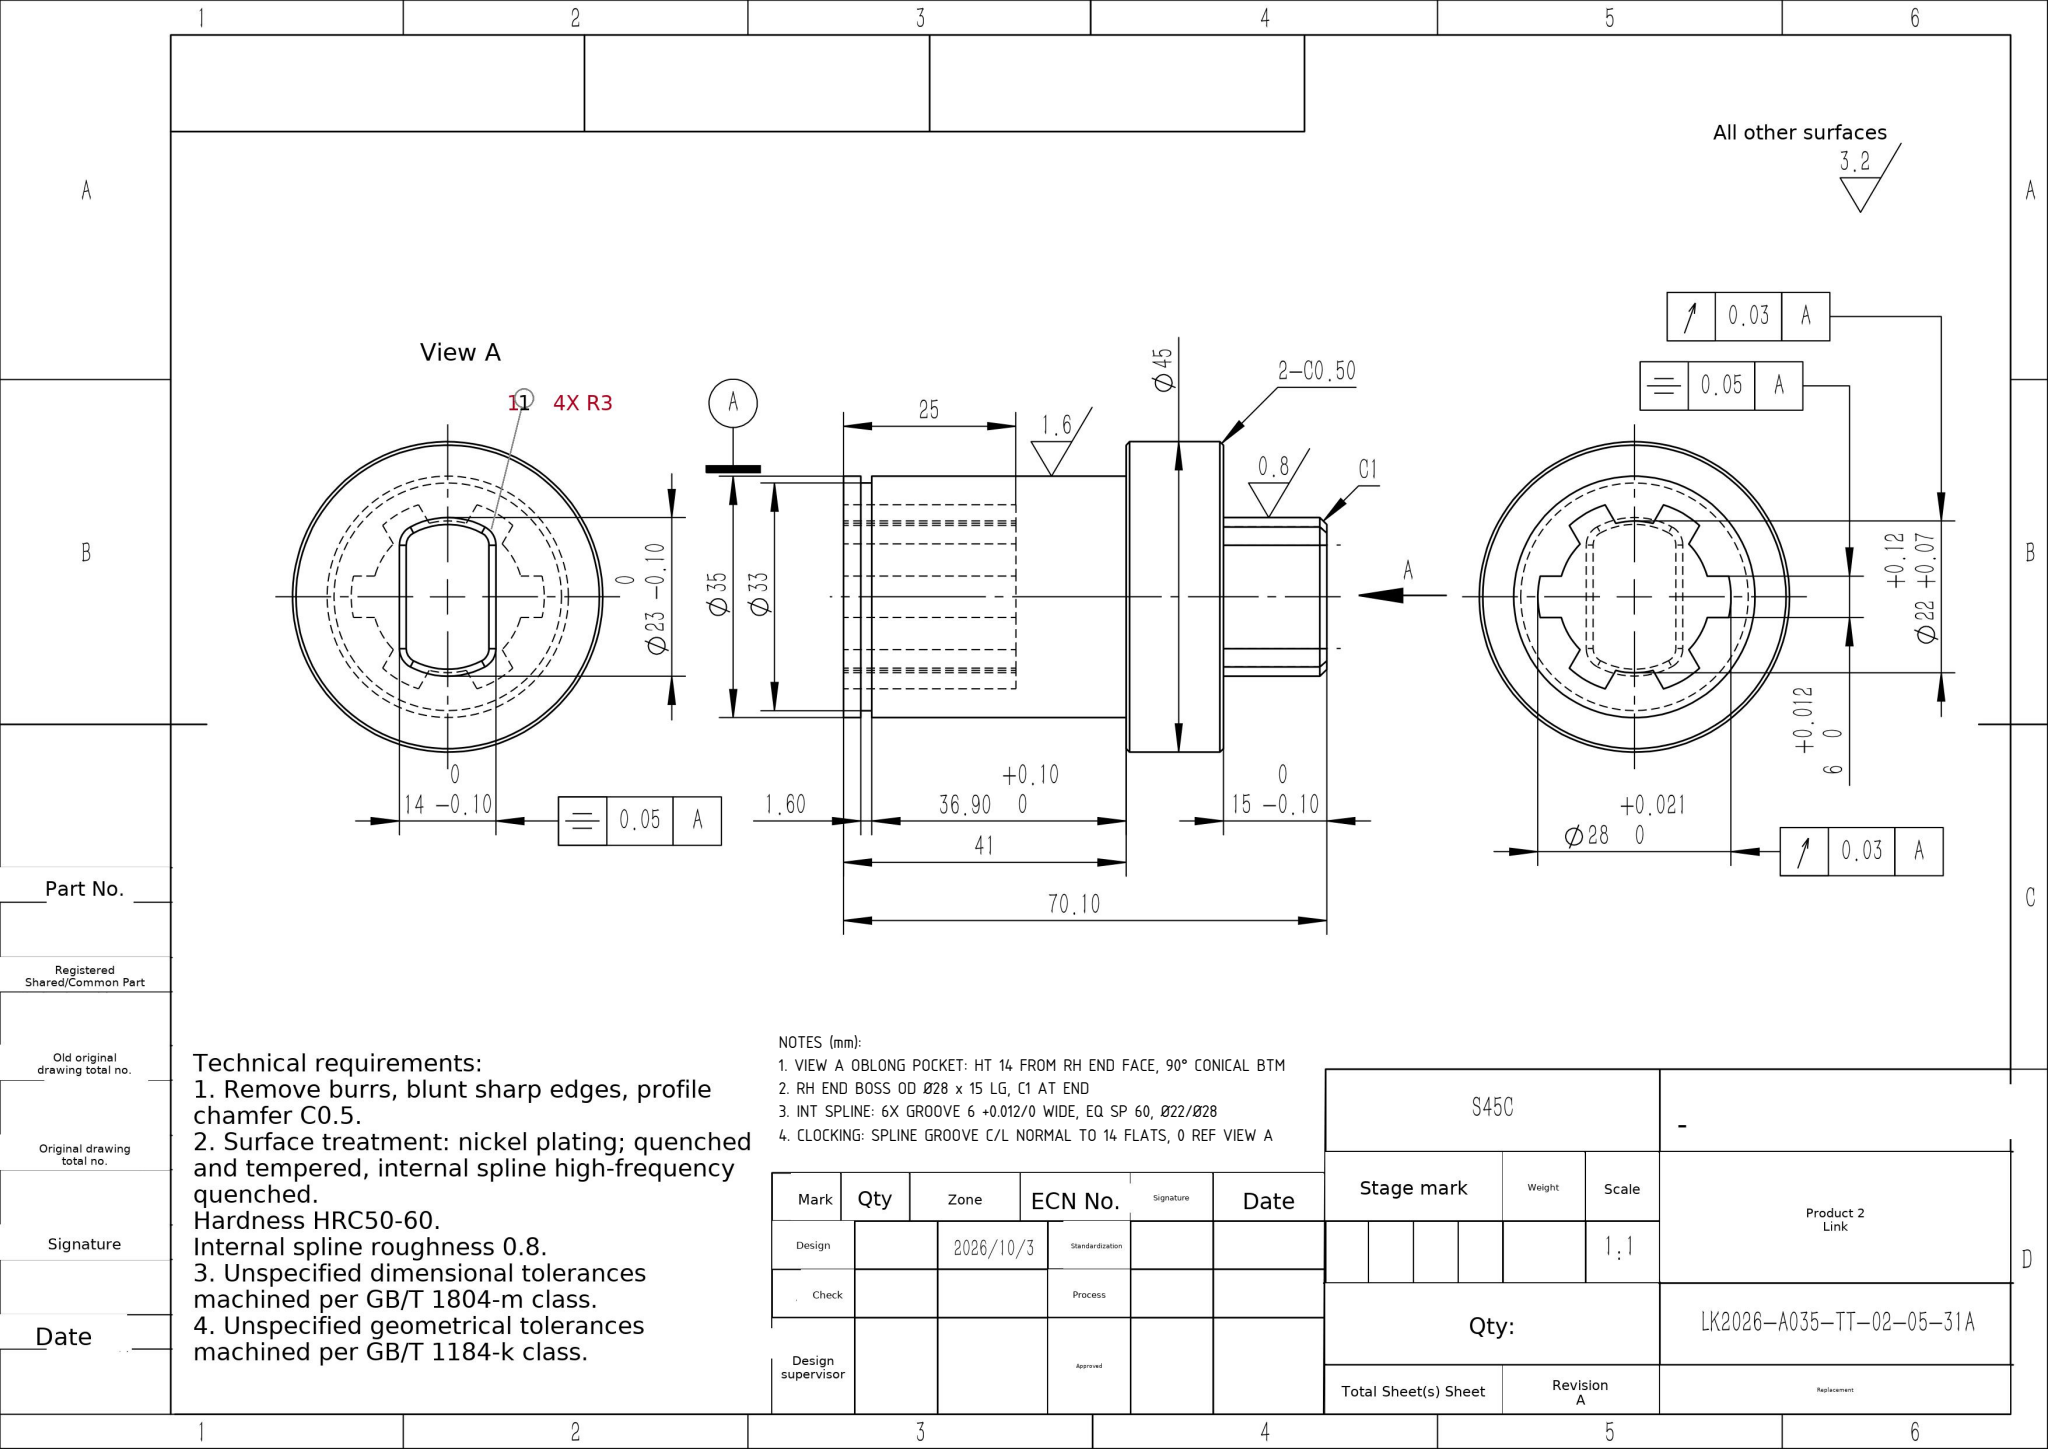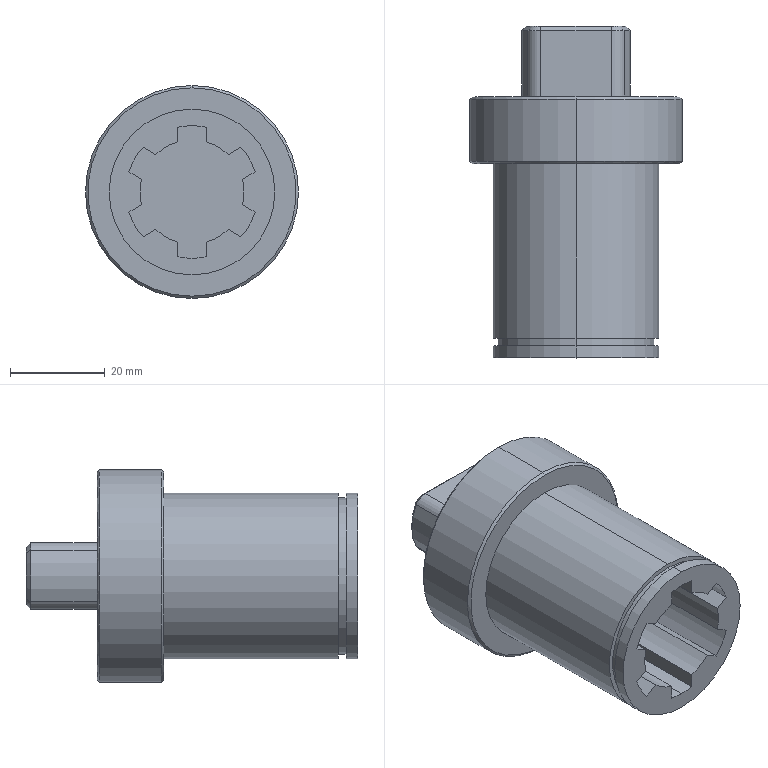Part | SolidWorks | mm | 1 solid | 60 faces | box 45 x 70.1 x 45 mm | volume 53889 mm3 | cylinder 27 | plane 23 | cone 10 | commonest cylinder face diameters 28 x7 22 x6 35 x4 6 x4 33 x2 45 x2 23 x2
Drawing notes:
VIEW A OBLONG POCKET: HT 14 FROM RH END FACE, 90° CONICAL BTM | from the solid: Ø23 cyl, axis y, L=14 from y=70.1 end face (boss face y=55.1-70.1); 4X Ø6 corner cyls L=14; cone 90° incl, ref dia 21 at pocket bottom
RH END BOSS OD Ø28 x 15 LG, C1 AT END | from the solid: Ø28 cyl group (count 7 = 6 spline major arcs + boss OD); boss between y-planes 55.1 and 70.1 = 15 lg, C1 chamfer at y=70.1
INT SPLINE: 6X GROOVE 6 +0.012/0 WIDE, EQ SP 60, Ø22/Ø28 | from the solid: Ø22 minor cyl count 6 + Ø28 major cyl; groove flanks at x=19.5 & 25.5 (6 apart) about axis x=22.5 -> 6 grooves eq sp 60 deg
CLOCKING: SPLINE GROOVE C/L NORMAL TO 14 FLATS, 0 REF VIEW A | from the solid: Pocket flats at z=15.5 & 29.5 (normal z, 14 apart); spline groove flanks x=19.5/25.5 symmetric about x=22.5, groove centered on +/-z axis
build123d program:
from build123d import *

# Parameters (mm, degrees)
CUT_EXTRUDE1_DEPTH  = 25
CHAMFER1_SIZE       = 0.5
SKETCH4_R           = 11.5
BOSS_EXTRUDE1_DEPTH = 15
SKETCH5_W           = 25
SKETCH5_H           = 9
CUT_EXTRUDE3_DEPTH  = 15
FILLET1_R           = 3
CHAMFER2_SIZE       = 1


with BuildPart() as part:
    # Sketch1 → Revolve1 (revolve)
    with BuildSketch(Plane(origin=(0, 0, 1073), x_dir=(-1, 0, 0), z_dir=(0, 0, -1)), mode=Mode.PRIVATE) as revolve1_sk:
        Polygon((-17.5, -55.1), (0, -55.1), (0, 0), (-22.5, 0), (-22.5, -14.1), (-17.5, -14.1), (-17.5, -51), (-16.5, -51), (-16.5, -52.6), (-17.5, -52.6), align=None)
    revolve(revolve1_sk.sketch.rotate(Axis((0, -55.1, 1073), (0, 1, 0)), 270), axis=Axis((0, -55.1, 1073), (0, 1, 0)))

    # Sketch2 → Cut-Extrude1 (cut)
    with BuildSketch(Plane.XZ.offset(55.1)):
        with BuildLine():
            Line((-3, 1086.675), (-3, 1083.583))
            ThreePointArc((-3, 1083.583), (-5.5, 1082.526), (-7.665, 1080.89))
            Line((-7.665, 1080.89), (-10.343, 1082.435))
            ThreePointArc((-10.343, 1082.435), (-12.124, 1080), (-13.343, 1077.239))
            Line((-13.343, 1077.239), (-10.665, 1075.693))
            ThreePointArc((-10.665, 1075.693), (-11, 1073), (-10.665, 1070.307))
            Line((-10.665, 1070.307), (-13.343, 1068.761))
            ThreePointArc((-13.343, 1068.761), (-12.124, 1066), (-10.343, 1063.565))
            Line((-10.343, 1063.565), (-7.665, 1065.11))
            ThreePointArc((-7.665, 1065.11), (-5.5, 1063.474), (-3, 1062.417))
            Line((-3, 1062.417), (-3, 1059.325))
            ThreePointArc((-3, 1059.325), (0, 1059), (3, 1059.325))
            Line((3, 1059.325), (3, 1062.417))
            ThreePointArc((3, 1062.417), (5.5, 1063.474), (7.665, 1065.11))
            Line((7.665, 1065.11), (10.343, 1063.565))
            ThreePointArc((10.343, 1063.565), (12.124, 1066), (13.343, 1068.761))
            Line((13.343, 1068.761), (10.665, 1070.307))
            ThreePointArc((10.665, 1070.307), (11, 1073), (10.665, 1075.693))
            Line((10.665, 1075.693), (13.343, 1077.239))
            ThreePointArc((13.343, 1077.239), (12.124, 1080), (10.343, 1082.435))
            Line((10.343, 1082.435), (7.665, 1080.89))
            ThreePointArc((7.665, 1080.89), (5.5, 1082.526), (3, 1083.583))
            Line((3, 1083.583), (3, 1086.675))
            ThreePointArc((3, 1086.675), (0, 1087), (-3, 1086.675))
        make_face()
    extrude(amount=-CUT_EXTRUDE1_DEPTH, mode=Mode.SUBTRACT)

    # Chamfer1
    chamfer1_edges = [part.edges().sort_by_distance(p)[0] for p in [
        (0, -14.1, 1050.5),
        (0, 0, 1050.5),
    ]]
    chamfer(chamfer1_edges, length=CHAMFER1_SIZE)

    # Sketch4 → Boss-Extrude1 (add)
    with BuildSketch(Plane(origin=(0, 0, 0), x_dir=(1, 0, 0), z_dir=(0, 1, 0))):
        with Locations(Location((0, -1073, 0), (0, 0, 270))):
            Circle(SKETCH4_R)
    extrude(amount=BOSS_EXTRUDE1_DEPTH)

    # Sketch5 → Cut-Extrude3 (cut)
    with BuildSketch(Plane(origin=(0, 15, 0), x_dir=(1, 0, 0), z_dir=(0, 1, 0))):
        with Locations((0, -1061.5)):
            Rectangle(SKETCH5_W, SKETCH5_H)
        with Locations((0, -1084.5)):
            Rectangle(SKETCH5_W, SKETCH5_H)
    extrude(amount=-CUT_EXTRUDE3_DEPTH, mode=Mode.SUBTRACT)

    # Fillet1
    fillet1_edges = [part.edges().sort_by_distance(p)[0] for p in [
        (-9.124, 7.5, 1066),
        (9.124, 7.5, 1066),
        (9.124, 7.5, 1080),
        (-9.124, 7.5, 1080),
    ]]
    fillet(fillet1_edges, radius=FILLET1_R)

    # Chamfer2
    chamfer2_edges = [part.edges().sort_by_distance(p)[0] for p in [
        (11.5, 15, 1073),
        (0, 15, 1066),
        (-11.5, 15, 1073),
        (0, 15, 1080),
        (-9.043, 15, 1079.572),
        (-9.043, 15, 1066.428),
        (9.043, 15, 1079.572),
        (9.043, 15, 1066.428),
    ]]
    chamfer(chamfer2_edges, length=CHAMFER2_SIZE)


solid = part.part